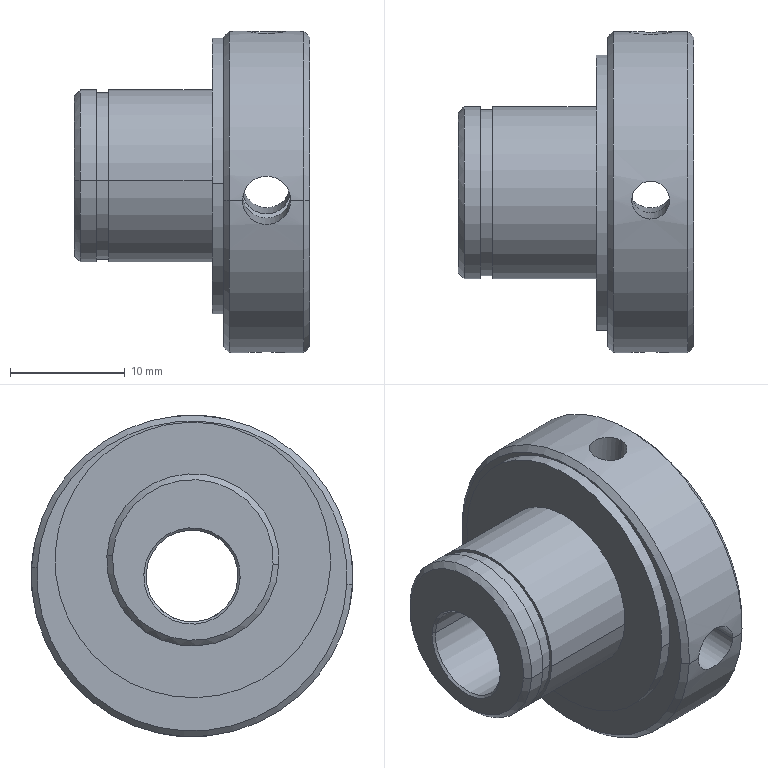Component | SolidWorks | EccentricWheel-1 | 1 solid | 36 faces | box 20.5 x 28 x 28 mm | volume 5613 mm3 | cylinder 20 | cone 10 | plane 6 | commonest cylinder face diameters 4.2 x6 15 x4 14.5 x2 24 x2 3.3 x2 8 x2 28 x2 | material GCr15
build123d program:
from build123d import *

# Parameters (mm, degrees)
SKETCH12_R               = 14
BOSS_EXTRUDE4_DEPTH      = 7.5
SKETCH13_R               = 7.5
BOSS_EXTRUDE5_DEPTH      = 13
F_5_0_5_DIAMETER_HOLE1_D = 8
SKETCH17_W               = 2.1
SKETCH17_H               = 14
M4_TAPPED_HOLE1_D        = 3.3
SKETCH21_W               = 2.1
SKETCH21_H               = 14
CHAMFER2_SIZE            = 0.2
SKETCH26_R               = 12
SKETCH26_R_2             = 7.5
BOSS_EXTRUDE6_DEPTH      = 1
CHAMFER3_SIZE            = 0.5
SKETCH27_R               = 7.5
SKETCH27_R_2             = 7.25
CUT_EXTRUDE1_DEPTH       = 1.1
M5_TAPPED_HOLE3_D        = 4.2


with BuildPart() as part:
    # Sketch12 → Boss-Extrude4 (new body)
    with BuildSketch(Plane.XY):
        Circle(SKETCH12_R)
    extrude(amount=BOSS_EXTRUDE4_DEPTH)

    # Sketch13 → Boss-Extrude5 (add)
    with BuildSketch(Plane.XY.offset(7.5)):
        with Locations(Location((0, -1.4, 0), (0, 0, 180))):
            Circle(SKETCH13_R)
    extrude(amount=BOSS_EXTRUDE5_DEPTH)

    # 5.0 _5_ Diameter Hole1 (through all)
    with Locations(Plane(origin=(0, 0, 0), x_dir=(-1, 0, 0), z_dir=(0, 0, -1))):
        with Locations((0, 0)):
            Hole(F_5_0_5_DIAMETER_HOLE1_D / 2)

    # Sketch17 → M5 Tapped Hole2 (revolve, cut)
    with BuildSketch(Plane(origin=(0, 0, 3.75), x_dir=(0, 0, -1), z_dir=(1, 0, 0))):
        with Locations((1.05, 7)):
            Rectangle(SKETCH17_W, SKETCH17_H)
    revolve(axis=Axis((0, -6.35, 3.75), (0, 1, 0)), mode=Mode.SUBTRACT)

    # M4 Tapped Hole1 (through all)
    with Locations(Plane(origin=(0, 0, 0), x_dir=(1, 0, 0), z_dir=(0, 1, 0))):
        with Locations((0, -3.75)):
            Hole(M4_TAPPED_HOLE1_D / 2)

    # Sketch21 → M5 Tapped Hole1 (revolve, cut)
    with BuildSketch(Plane(origin=(0, 0, 3.75), x_dir=(0, 0, -1), z_dir=(0, 1, 0))):
        with Locations((1.05, 7)):
            Rectangle(SKETCH21_W, SKETCH21_H)
    revolve(axis=Axis((6.35, 0, 3.75), (-1, 0, 0)), mode=Mode.SUBTRACT)

    # Chamfer2
    chamfer2_edges = [part.edges().sort_by_distance(p)[0] for p in [
        (-4, 0, 0),
        (-4, 0, 20.5),
    ]]
    chamfer(chamfer2_edges, length=CHAMFER2_SIZE)

    # Sketch26 → Boss-Extrude6 (add)
    with BuildSketch(Plane.XY.offset(7.5)):
        with Locations((0, -1.4)):
            Circle(SKETCH26_R)
        with Locations(Location((0, -1.4, 0), (0, 0, 180))):
            Circle(SKETCH26_R_2, mode=Mode.SUBTRACT)
    extrude(amount=BOSS_EXTRUDE6_DEPTH)

    # Chamfer3
    chamfer3_edges = [part.edges().sort_by_distance(p)[0] for p in [
        (-14, 0, 0),
        (-14, 0, 7.5),
        (7.5, -1.4, 20.5),
    ]]
    chamfer(chamfer3_edges, length=CHAMFER3_SIZE)

    # Sketch27 → Cut-Extrude1 (cut)
    with BuildSketch(Plane.XY.offset(17.5)):
        with Locations(Location((0, -1.4, 0), (0, 0, 180))):
            Circle(SKETCH27_R)
        with Locations((0, -1.4)):
            Circle(SKETCH27_R_2, mode=Mode.SUBTRACT)
    extrude(amount=CUT_EXTRUDE1_DEPTH, mode=Mode.SUBTRACT)

    # M5 Tapped Hole3 (through all)
    with Locations(Plane(origin=(0, 0, 0), x_dir=(0, 0, -1), z_dir=(-1, 0, 0))):
        with Locations((-3.75, 0)):
            Hole(M5_TAPPED_HOLE3_D / 2)


solid = part.part

# Placed as in the assembly
solid = solid.moved(Location((18.226, -5.336, 80.465), (-111.257, -89.998, -24.271)))